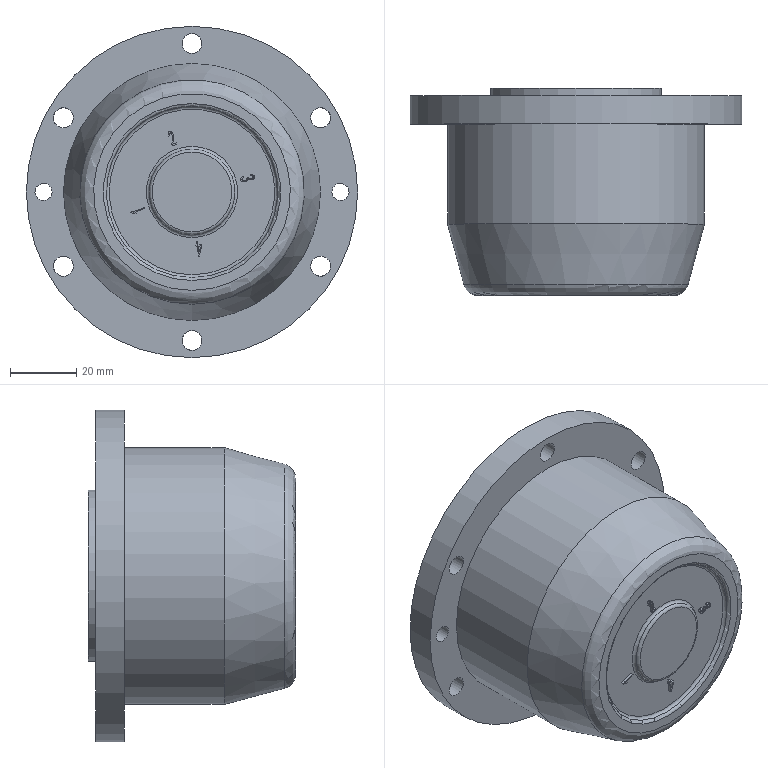Component | NX | MOTOR | 1 solid | 96 faces | volume 295247 mm3 | other 41 | plane 38 | cylinder 11 | torus 5 | cone 1 | commonest cylinder face diameters 6.02 x6 5.16 x2 99.76 x1 77.4 x1 51.6 x1